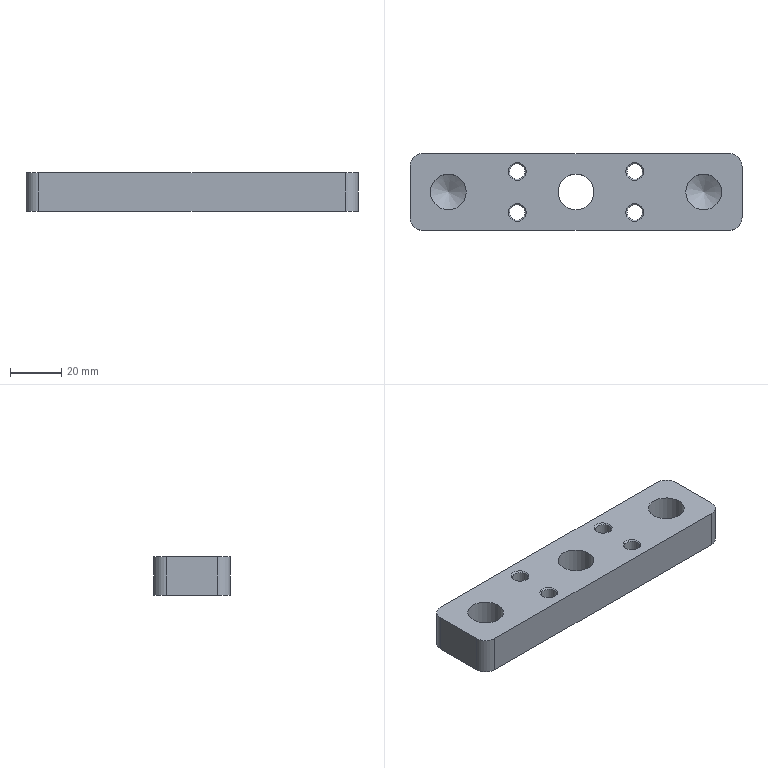Component | NX | V_BLOCK_FIX_PLATE | 1 solid | 23 faces | volume 50652 mm3 | cylinder 11 | plane 6 | cone 6 | commonest cylinder face diameters 10 x4 6 x4 14 x3